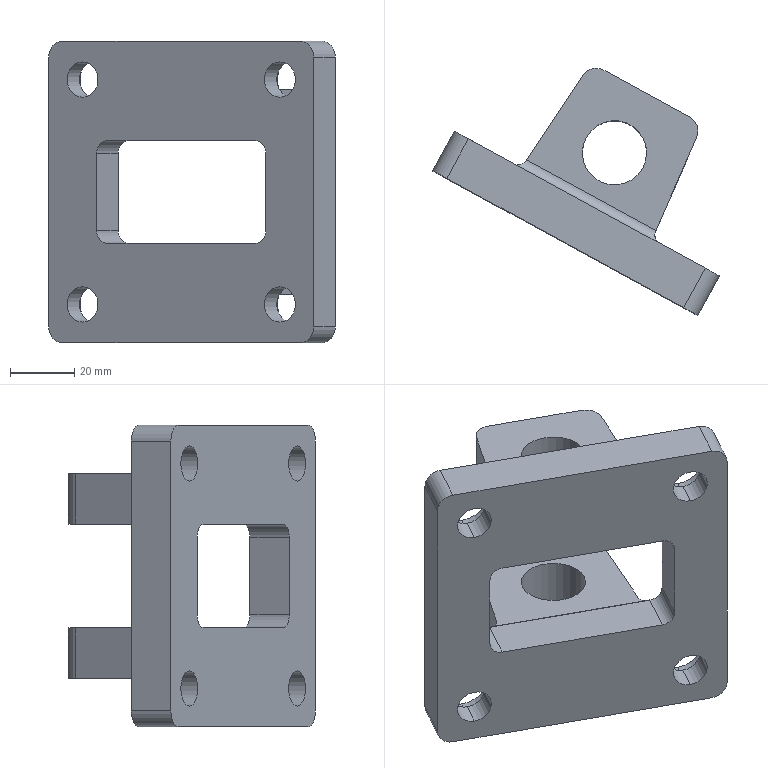Component | SolidWorks | CB-80CylinderFixingBase(DoubleEyelet)-1 | 1 solid | 62 faces | box 89.22 x 76.92 x 94 mm | volume 131345 mm3 | cylinder 38 | plane 24 | commonest cylinder face diameters 17 x8 11 x8 10 x8 6 x6 20 x4 8 x4
build123d program:
from build123d import *

# Parameters (mm, degrees)
SKETCH1_W                                            = 94
SKETCH1_H                                            = 94
SKETCH1_W_2                                          = 60
SKETCH1_H_2                                          = 32
BOSS_EXTRUDE1_DEPTH                                  = 14
FILLET1_R                                            = 5
FILLET2_R                                            = 4
CYLINDRICAL_COUNTERSUNK_HOLE_FOR_M10_HEX_D           = 11
CYLINDRICAL_COUNTERSUNK_HOLE_FOR_M10_HEX_CBORE_D     = 17
CYLINDRICAL_COUNTERSUNK_HOLE_FOR_M10_HEX_CBORE_DEPTH = 6
LPATTERN1_COUNT                                      = 2
LPATTERN1_PITCH                                      = 70
LPATTERN1_COUNT_DIR2                                 = 2
LPATTERN1_PITCH_DIR2                                 = 70
SKETCH5_W                                            = 46.336
SKETCH5_H                                            = 15.85
BOSS_EXTRUDE2_DEPTH                                  = 39
DRAFT1_ANGLE                                         = 5
DRAFT1_OF_MIRROR1_2_ANGLE                            = 5
SKETCH6_R                                            = 10
CUT_EXTRUDE1_DEPTH                                   = 34.5
FILLET3_R                                            = 5
FILLET4_R                                            = 3


with BuildPart() as part:
    # Sketch1 → Boss-Extrude1 (new body)
    with BuildSketch(Plane(origin=(0, 0, 0), x_dir=(1, 0, 0), z_dir=(0, 1, 0))):
        Rectangle(SKETCH1_W, SKETCH1_H)
        Rectangle(SKETCH1_W_2, SKETCH1_H_2, mode=Mode.SUBTRACT)
    extrude(amount=BOSS_EXTRUDE1_DEPTH)

    # Fillet1
    fillet1_edges = [part.edges().sort_by_distance(p)[0] for p in [
        (47, 7, 47),
        (-47, 7, 47),
        (-47, 7, -47),
        (47, 7, -47),
    ]]
    fillet(fillet1_edges, radius=FILLET1_R)

    # Fillet2
    fillet2_edges = [part.edges().sort_by_distance(p)[0] for p in [
        (30, 7, 16),
        (30, 7, -16),
        (-30, 7, -16),
        (-30, 7, 16),
    ]]
    fillet(fillet2_edges, radius=FILLET2_R)

    # Cylindrical Countersunk Hole for M10 Hex (through all)
    with Locations(Plane(origin=(0, 14, 0), x_dir=(1, 0, 0), z_dir=(0, 1, 0))):
        with Locations((-35, 35)):
            cylindrical_countersunk_hole_for_m10_hex = CounterBoreHole(CYLINDRICAL_COUNTERSUNK_HOLE_FOR_M10_HEX_D / 2, CYLINDRICAL_COUNTERSUNK_HOLE_FOR_M10_HEX_CBORE_D / 2, CYLINDRICAL_COUNTERSUNK_HOLE_FOR_M10_HEX_CBORE_DEPTH)

    # LPattern1: Cylindrical Countersunk Hole for M10 Hex 2 × 2
    with Locations(*[(j * LPATTERN1_PITCH_DIR2, 0, i * LPATTERN1_PITCH) for i in range(LPATTERN1_COUNT) for j in range(LPATTERN1_COUNT_DIR2) if (i, j) != (0, 0)]):
        add(cylindrical_countersunk_hole_for_m10_hex, mode=Mode.SUBTRACT)

    # Sketch5 → Boss-Extrude2 (add)
    with BuildSketch(Plane(origin=(0, 14, 0), x_dir=(1, 0, 0), z_dir=(0, 1, 0))):
        with Locations((0, 24.075)):
            Rectangle(SKETCH5_W, SKETCH5_H)
    boss_extrude2 = extrude(amount=BOSS_EXTRUDE2_DEPTH)

    # Draft1
    draft1_faces = [part.faces().sort_by_distance(p)[0] for p in [
        (23.168, 33.5, -24.075),
        (-23.168, 33.5, -24.075),
    ]]
    draft(draft1_faces, Plane.ZX.offset(14), DRAFT1_ANGLE)

    # Mirror1: Boss-Extrude2 across plane
    add(boss_extrude2.mirror(Plane.XY))

    # Draft1 of Mirror1 2
    draft1_of_mirror1_2_faces = [part.faces().sort_by_distance(p)[0] for p in [
        (23.168, 33.5, 24.075),
        (-23.168, 33.5, 24.075),
    ]]
    draft(draft1_of_mirror1_2_faces, Plane(origin=(0, 14, 0), x_dir=(0, 0, -1), z_dir=(0, 1, 0)), DRAFT1_OF_MIRROR1_2_ANGLE)

    # Sketch6 → Cut-Extrude1 (cut, symmetric)
    with BuildSketch(Plane.XY):
        with Locations((0, 32)):
            Circle(SKETCH6_R)
    extrude(amount=CUT_EXTRUDE1_DEPTH, both=True, mode=Mode.SUBTRACT)

    # Fillet3
    fillet3_edges = [part.edges().sort_by_distance(p)[0] for p in [
        (-19.756, 53, -24.075),
        (19.756, 53, -24.075),
        (-19.756, 53, 24.075),
        (19.756, 53, 24.075),
    ]]
    fillet(fillet3_edges, radius=FILLET3_R)

    # Fillet4
    fillet4_edges = [part.edges().sort_by_distance(p)[0] for p in [
        (-23.168, 14, -24.075),
        (23.168, 14, -24.075),
        (0, 14, -32),
        (-23.168, 14, 24.075),
        (23.168, 14, 24.075),
        (0, 14, 32),
    ]]
    fillet(fillet4_edges, radius=FILLET4_R)


solid = part.part

# Placed as in the assembly
solid = solid.moved(Location((-148.101, 368.145, 900), (180, 0, -151.378)))